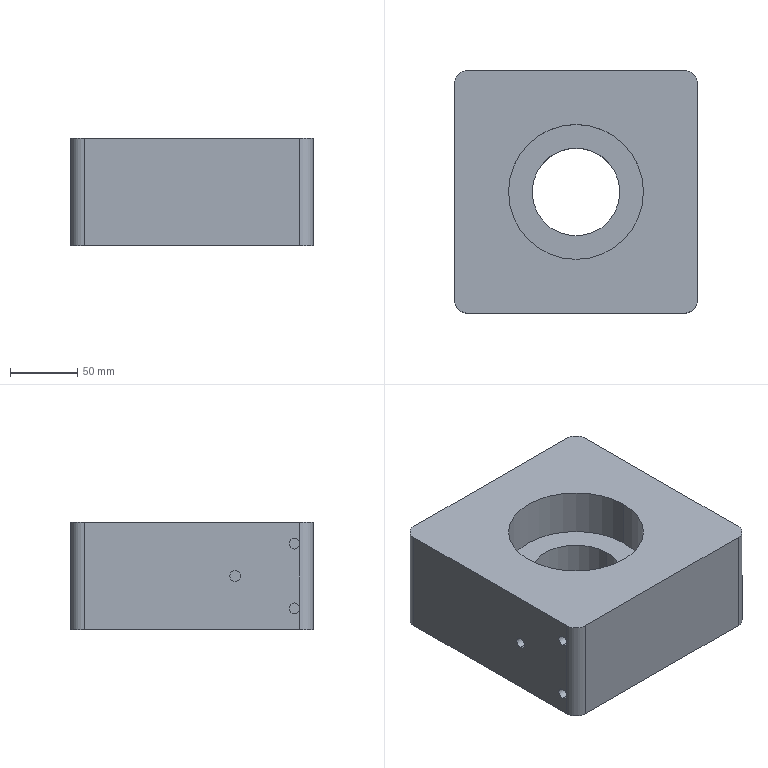Component | SolidWorks | CleaningRobotAssembly-1_FixingBlock-1 | 1 solid | 33 faces | box 180 x 180 x 80 mm | volume 2157904 mm3 | cylinder 20 | plane 13 | commonest cylinder face diameters 8 x12 20 x4 100 x2 65 x2
build123d program:
from build123d import *

# Parameters (mm, degrees)
SKETCH1_W           = 180
SKETCH1_H           = 180
BOSS_EXTRUDE1_DEPTH = 80
SKETCH2_R           = 32.5
CUT_EXTRUDE1_DEPTH  = 100
FILLET1_R           = 10
SKETCH3_R           = 4
CUT_EXTRUDE2_DEPTH  = 10
SKETCH4_R           = 50
CUT_EXTRUDE3_DEPTH  = 35


with BuildPart() as part:
    # Sketch1 → Boss-Extrude1 (new body)
    with BuildSketch(Plane.XY):
        Rectangle(SKETCH1_W, SKETCH1_H)
    extrude(amount=BOSS_EXTRUDE1_DEPTH)

    # Sketch2 → Cut-Extrude1 (cut)
    with BuildSketch(Plane(origin=(0, 0, 0), x_dir=(-1, 0, 0), z_dir=(0, 0, -1))):
        Circle(SKETCH2_R)
    extrude(amount=-CUT_EXTRUDE1_DEPTH, mode=Mode.SUBTRACT)

    # Fillet1
    fillet1_edges = [part.edges().sort_by_distance(p)[0] for p in [
        (-90, 90, 40),
        (90, 90, 40),
        (90, -90, 40),
        (-90, -90, 40),
    ]]
    fillet(fillet1_edges, radius=FILLET1_R)

    # Sketch3 → Cut-Extrude2 (cut)
    with BuildSketch(Plane(origin=(90, 0, 0), x_dir=(0, 0, -1), z_dir=(1, 0, 0))):
        with Locations((-16, 76)):
            Circle(SKETCH3_R)
        with Locations((-40, 32)):
            Circle(SKETCH3_R)
        with Locations((-64, 76)):
            Circle(SKETCH3_R)
    cut_extrude2 = extrude(amount=-CUT_EXTRUDE2_DEPTH, mode=Mode.SUBTRACT)

    # Mirror1: Cut-Extrude2 across plane
    add(cut_extrude2.mirror(Plane(origin=(0, 0, 0), x_dir=(0, 0, 1), z_dir=(1, 0, 0))), mode=Mode.SUBTRACT)

    # Sketch4 → Cut-Extrude3 (cut)
    with BuildSketch(Plane(origin=(0, 0, 0), x_dir=(-1, 0, 0), z_dir=(0, 0, -1))):
        Circle(SKETCH4_R)
    extrude(amount=-CUT_EXTRUDE3_DEPTH, mode=Mode.SUBTRACT)


solid = part.part

# Placed as in the assembly
solid = solid.moved(Location((310.629, 34.1, 268), (180, 0, 0)))
STEP:
#1=COLOUR_RGB('',0.7922,0.8196,0.9333);
#2=FILL_AREA_STYLE_COLOUR('',#1);
#3=FILL_AREA_STYLE('',(#2));
#4=SURFACE_STYLE_FILL_AREA(#3);
#5=SURFACE_SIDE_STYLE('',(#4));
#6=SURFACE_STYLE_USAGE(.BOTH.,#5);
#7=PRESENTATION_STYLE_ASSIGNMENT((#6));
#8=CARTESIAN_POINT('',(14.198,1.343,9.173));
#9=VERTEX_POINT('',#8);
#10=CARTESIAN_POINT('',(10.261,1.343,9.173));
#11=VERTEX_POINT('',#10);
#12=CARTESIAN_POINT('',(12.23,1.343,9.173));
#13=DIRECTION('',(0.,0.,1.));
#14=DIRECTION('',(-1.,-0.,0.));
#15=AXIS2_PLACEMENT_3D('',#12,#13,#14);
#16=CIRCLE('',#15,1.969);
#17=EDGE_CURVE('',#9,#11,#16,.T.);
#18=ORIENTED_EDGE('',*,*,#17,.F.);
#19=CARTESIAN_POINT('',(14.198,1.343,10.551));
#20=VERTEX_POINT('',#19);
#21=CARTESIAN_POINT('',(14.198,1.343,9.173));
#22=DIRECTION('',(0.,0.,1.));
#23=VECTOR('',#22,39.37);
#24=LINE('',#21,#23);
#25=EDGE_CURVE('',#9,#20,#24,.T.);
#26=ORIENTED_EDGE('',*,*,#25,.T.);
#27=CARTESIAN_POINT('',(10.261,1.343,10.551));
#28=VERTEX_POINT('',#27);
#29=CARTESIAN_POINT('',(12.23,1.343,10.551));
#30=DIRECTION('',(0.,0.,1.));
#31=DIRECTION('',(-1.,-0.,0.));
#32=AXIS2_PLACEMENT_3D('',#29,#30,#31);
#33=CIRCLE('',#32,1.969);
#34=EDGE_CURVE('',#20,#28,#33,.T.);
#35=ORIENTED_EDGE('',*,*,#34,.T.);
#36=CARTESIAN_POINT('',(10.261,1.343,9.173));
#37=DIRECTION('',(0.,0.,1.));
#38=VECTOR('',#37,39.37);
#39=LINE('',#36,#38);
#40=EDGE_CURVE('',#11,#28,#39,.T.);
#41=ORIENTED_EDGE('',*,*,#40,.F.);
#42=EDGE_LOOP('',(#18,#26,#35,#41));
#43=FACE_OUTER_BOUND('',#42,.T.);
#44=CARTESIAN_POINT('',(12.23,1.343,9.173));
#45=DIRECTION('',(0.,0.,1.));
#46=DIRECTION('',(-1.,-0.,0.));
#47=AXIS2_PLACEMENT_3D('',#44,#45,#46);
#48=CYLINDRICAL_SURFACE('',#47,1.969);
#49=ADVANCED_FACE('',(#43),#48,.F.);
#50=CARTESIAN_POINT('',(9.08,-1.65,9.764));
#51=VERTEX_POINT('',#50);
#52=CARTESIAN_POINT('',(9.08,-1.65,10.079));
#53=VERTEX_POINT('',#52);
#54=CARTESIAN_POINT('',(9.08,-1.65,9.921));
#55=DIRECTION('',(1.,0.,-0.));
#56=DIRECTION('',(0.,0.,1.));
#57=AXIS2_PLACEMENT_3D('',#54,#55,#56);
#58=CIRCLE('',#57,0.1575);
#59=EDGE_CURVE('',#51,#53,#58,.T.);
#60=ORIENTED_EDGE('',*,*,#59,.T.);
#61=CARTESIAN_POINT('',(8.686,-1.65,10.079));
#62=VERTEX_POINT('',#61);
#63=CARTESIAN_POINT('',(9.08,-1.65,10.079));
#64=DIRECTION('',(-1.,-0.,0.));
#65=VECTOR('',#64,39.37);
#66=LINE('',#63,#65);
#67=EDGE_CURVE('',#53,#62,#66,.T.);
#68=ORIENTED_EDGE('',*,*,#67,.T.);
#69=CARTESIAN_POINT('',(8.686,-1.65,9.764));
#70=VERTEX_POINT('',#69);
#71=CARTESIAN_POINT('',(8.686,-1.65,9.921));
#72=DIRECTION('',(1.,0.,-0.));
#73=DIRECTION('',(0.,0.,1.));
#74=AXIS2_PLACEMENT_3D('',#71,#72,#73);
#75=CIRCLE('',#74,0.1575);
#76=EDGE_CURVE('',#70,#62,#75,.T.);
#77=ORIENTED_EDGE('',*,*,#76,.F.);
#78=CARTESIAN_POINT('',(9.08,-1.65,9.764));
#79=DIRECTION('',(-1.,-0.,0.));
#80=VECTOR('',#79,39.37);
#81=LINE('',#78,#80);
#82=EDGE_CURVE('',#51,#70,#81,.T.);
#83=ORIENTED_EDGE('',*,*,#82,.F.);
#84=EDGE_LOOP('',(#60,#68,#77,#83));
#85=FACE_OUTER_BOUND('',#84,.T.);
#86=CARTESIAN_POINT('',(9.08,-1.65,9.921));
#87=DIRECTION('',(-1.,-0.,0.));
#88=DIRECTION('',(0.,0.,-1.));
#89=AXIS2_PLACEMENT_3D('',#86,#87,#88);
#90=CYLINDRICAL_SURFACE('',#89,0.1575);
#91=ADVANCED_FACE('',(#85),#90,.F.);
#92=CARTESIAN_POINT('',(9.08,0.08267,8.819));
#93=VERTEX_POINT('',#92);
#94=CARTESIAN_POINT('',(9.08,0.08267,9.134));
#95=VERTEX_POINT('',#94);
#96=CARTESIAN_POINT('',(9.08,0.08267,8.976));
#97=DIRECTION('',(1.,0.,-0.));
#98=DIRECTION('',(0.,0.,1.));
#99=AXIS2_PLACEMENT_3D('',#96,#97,#98);
#100=CIRCLE('',#99,0.1575);
#101=EDGE_CURVE('',#93,#95,#100,.T.);
#102=ORIENTED_EDGE('',*,*,#101,.T.);
#103=CARTESIAN_POINT('',(8.686,0.08267,9.134));
#104=VERTEX_POINT('',#103);
#105=CARTESIAN_POINT('',(9.08,0.08267,9.134));
#106=DIRECTION('',(-1.,-0.,0.));
#107=VECTOR('',#106,39.37);
#108=LINE('',#105,#107);
#109=EDGE_CURVE('',#95,#104,#108,.T.);
#110=ORIENTED_EDGE('',*,*,#109,.T.);
#111=CARTESIAN_POINT('',(8.686,0.08267,8.819));
#112=VERTEX_POINT('',#111);
#113=CARTESIAN_POINT('',(8.686,0.08267,8.976));
#114=DIRECTION('',(1.,0.,-0.));
#115=DIRECTION('',(0.,0.,1.));
#116=AXIS2_PLACEMENT_3D('',#113,#114,#115);
#117=CIRCLE('',#116,0.1575);
#118=EDGE_CURVE('',#112,#104,#117,.T.);
#119=ORIENTED_EDGE('',*,*,#118,.F.);
#120=CARTESIAN_POINT('',(9.08,0.08267,8.819));
#121=DIRECTION('',(-1.,-0.,0.));
#122=VECTOR('',#121,39.37);
#123=LINE('',#120,#122);
#124=EDGE_CURVE('',#93,#112,#123,.T.);
#125=ORIENTED_EDGE('',*,*,#124,.F.);
#126=EDGE_LOOP('',(#102,#110,#119,#125));
#127=FACE_OUTER_BOUND('',#126,.T.);
#128=CARTESIAN_POINT('',(9.08,0.08267,8.976));
#129=DIRECTION('',(-1.,-0.,0.));
#130=DIRECTION('',(0.,0.,-1.));
#131=AXIS2_PLACEMENT_3D('',#128,#129,#130);
#132=CYLINDRICAL_SURFACE('',#131,0.1575);
#133=ADVANCED_FACE('',(#127),#132,.F.);
#134=CARTESIAN_POINT('',(9.08,-1.65,7.874));
#135=VERTEX_POINT('',#134);
#136=CARTESIAN_POINT('',(9.08,-1.65,8.189));
#137=VERTEX_POINT('',#136);
#138=CARTESIAN_POINT('',(9.08,-1.65,8.031));
#139=DIRECTION('',(1.,0.,-0.));
#140=DIRECTION('',(0.,0.,1.));
#141=AXIS2_PLACEMENT_3D('',#138,#139,#140);
#142=CIRCLE('',#141,0.1575);
#143=EDGE_CURVE('',#135,#137,#142,.T.);
#144=ORIENTED_EDGE('',*,*,#143,.T.);
#145=CARTESIAN_POINT('',(8.686,-1.65,8.189));
#146=VERTEX_POINT('',#145);
#147=CARTESIAN_POINT('',(9.08,-1.65,8.189));
#148=DIRECTION('',(-1.,-0.,0.));
#149=VECTOR('',#148,39.37);
#150=LINE('',#147,#149);
#151=EDGE_CURVE('',#137,#146,#150,.T.);
#152=ORIENTED_EDGE('',*,*,#151,.T.);
#153=CARTESIAN_POINT('',(8.686,-1.65,7.874));
#154=VERTEX_POINT('',#153);
#155=CARTESIAN_POINT('',(8.686,-1.65,8.031));
#156=DIRECTION('',(1.,0.,-0.));
#157=DIRECTION('',(0.,0.,1.));
#158=AXIS2_PLACEMENT_3D('',#155,#156,#157);
#159=CIRCLE('',#158,0.1575);
#160=EDGE_CURVE('',#154,#146,#159,.T.);
#161=ORIENTED_EDGE('',*,*,#160,.F.);
#162=CARTESIAN_POINT('',(9.08,-1.65,7.874));
#163=DIRECTION('',(-1.,-0.,0.));
#164=VECTOR('',#163,39.37);
#165=LINE('',#162,#164);
#166=EDGE_CURVE('',#135,#154,#165,.T.);
#167=ORIENTED_EDGE('',*,*,#166,.F.);
#168=EDGE_LOOP('',(#144,#152,#161,#167));
#169=FACE_OUTER_BOUND('',#168,.T.);
#170=CARTESIAN_POINT('',(9.08,-1.65,8.031));
#171=DIRECTION('',(-1.,-0.,0.));
#172=DIRECTION('',(0.,0.,-1.));
#173=AXIS2_PLACEMENT_3D('',#170,#171,#172);
#174=CYLINDRICAL_SURFACE('',#173,0.1575);
#175=ADVANCED_FACE('',(#169),#174,.F.);
#176=CARTESIAN_POINT('',(15.379,-1.65,9.764));
#177=VERTEX_POINT('',#176);
#178=CARTESIAN_POINT('',(15.379,-1.65,10.079));
#179=VERTEX_POINT('',#178);
#180=CARTESIAN_POINT('',(15.379,-1.65,9.921));
#181=DIRECTION('',(1.,0.,-0.));
#182=DIRECTION('',(0.,0.,1.));
#183=AXIS2_PLACEMENT_3D('',#180,#181,#182);
#184=CIRCLE('',#183,0.1575);
#185=EDGE_CURVE('',#177,#179,#184,.T.);
#186=ORIENTED_EDGE('',*,*,#185,.F.);
#187=CARTESIAN_POINT('',(15.773,-1.65,9.764));
#188=VERTEX_POINT('',#187);
#189=CARTESIAN_POINT('',(15.379,-1.65,9.764));
#190=DIRECTION('',(1.,0.,-0.));
#191=VECTOR('',#190,39.37);
#192=LINE('',#189,#191);
#193=EDGE_CURVE('',#177,#188,#192,.T.);
#194=ORIENTED_EDGE('',*,*,#193,.T.);
#195=CARTESIAN_POINT('',(15.773,-1.65,10.079));
#196=VERTEX_POINT('',#195);
#197=CARTESIAN_POINT('',(15.773,-1.65,9.921));
#198=DIRECTION('',(1.,0.,-0.));
#199=DIRECTION('',(0.,0.,1.));
#200=AXIS2_PLACEMENT_3D('',#197,#198,#199);
#201=CIRCLE('',#200,0.1575);
#202=EDGE_CURVE('',#188,#196,#201,.T.);
#203=ORIENTED_EDGE('',*,*,#202,.T.);
#204=CARTESIAN_POINT('',(15.379,-1.65,10.079));
#205=DIRECTION('',(1.,0.,-0.));
#206=VECTOR('',#205,39.37);
#207=LINE('',#204,#206);
#208=EDGE_CURVE('',#179,#196,#207,.T.);
#209=ORIENTED_EDGE('',*,*,#208,.F.);
#210=EDGE_LOOP('',(#186,#194,#203,#209));
#211=FACE_OUTER_BOUND('',#210,.T.);
#212=CARTESIAN_POINT('',(15.379,-1.65,9.921));
#213=DIRECTION('',(1.,0.,-0.));
#214=DIRECTION('',(0.,0.,1.));
#215=AXIS2_PLACEMENT_3D('',#212,#213,#214);
#216=CYLINDRICAL_SURFACE('',#215,0.1575);
#217=ADVANCED_FACE('',(#211),#216,.F.);
#218=CARTESIAN_POINT('',(15.379,0.08267,8.819));
#219=VERTEX_POINT('',#218);
#220=CARTESIAN_POINT('',(15.379,0.08267,9.134));
#221=VERTEX_POINT('',#220);
#222=CARTESIAN_POINT('',(15.379,0.08267,8.976));
#223=DIRECTION('',(1.,0.,-0.));
#224=DIRECTION('',(0.,0.,1.));
#225=AXIS2_PLACEMENT_3D('',#222,#223,#224);
#226=CIRCLE('',#225,0.1575);
#227=EDGE_CURVE('',#219,#221,#226,.T.);
#228=ORIENTED_EDGE('',*,*,#227,.F.);
#229=CARTESIAN_POINT('',(15.773,0.08267,8.819));
#230=VERTEX_POINT('',#229);
#231=CARTESIAN_POINT('',(15.379,0.08267,8.819));
#232=DIRECTION('',(1.,0.,-0.));
#233=VECTOR('',#232,39.37);
#234=LINE('',#231,#233);
#235=EDGE_CURVE('',#219,#230,#234,.T.);
#236=ORIENTED_EDGE('',*,*,#235,.T.);
#237=CARTESIAN_POINT('',(15.773,0.08267,9.134));
#238=VERTEX_POINT('',#237);
#239=CARTESIAN_POINT('',(15.773,0.08267,8.976));
#240=DIRECTION('',(1.,0.,-0.));
#241=DIRECTION('',(0.,0.,1.));
#242=AXIS2_PLACEMENT_3D('',#239,#240,#241);
#243=CIRCLE('',#242,0.1575);
#244=EDGE_CURVE('',#230,#238,#243,.T.);
#245=ORIENTED_EDGE('',*,*,#244,.T.);
#246=CARTESIAN_POINT('',(15.379,0.08267,9.134));
#247=DIRECTION('',(1.,0.,-0.));
#248=VECTOR('',#247,39.37);
#249=LINE('',#246,#248);
#250=EDGE_CURVE('',#221,#238,#249,.T.);
#251=ORIENTED_EDGE('',*,*,#250,.F.);
#252=EDGE_LOOP('',(#228,#236,#245,#251));
#253=FACE_OUTER_BOUND('',#252,.T.);
#254=CARTESIAN_POINT('',(15.379,0.08267,8.976));
#255=DIRECTION('',(1.,0.,-0.));
#256=DIRECTION('',(0.,0.,1.));
#257=AXIS2_PLACEMENT_3D('',#254,#255,#256);
#258=CYLINDRICAL_SURFACE('',#257,0.1575);
#259=ADVANCED_FACE('',(#253),#258,.F.);
#260=CARTESIAN_POINT('',(15.379,-1.65,7.874));
#261=VERTEX_POINT('',#260);
#262=CARTESIAN_POINT('',(15.379,-1.65,8.189));
#263=VERTEX_POINT('',#262);
#264=CARTESIAN_POINT('',(15.379,-1.65,8.031));
#265=DIRECTION('',(1.,0.,-0.));
#266=DIRECTION('',(0.,0.,1.));
#267=AXIS2_PLACEMENT_3D('',#264,#265,#266);
#268=CIRCLE('',#267,0.1575);
#269=EDGE_CURVE('',#261,#263,#268,.T.);
#270=ORIENTED_EDGE('',*,*,#269,.F.);
#271=CARTESIAN_POINT('',(15.773,-1.65,7.874));
#272=VERTEX_POINT('',#271);
#273=CARTESIAN_POINT('',(15.379,-1.65,7.874));
#274=DIRECTION('',(1.,0.,-0.));
#275=VECTOR('',#274,39.37);
#276=LINE('',#273,#275);
#277=EDGE_CURVE('',#261,#272,#276,.T.);
#278=ORIENTED_EDGE('',*,*,#277,.T.);
#279=CARTESIAN_POINT('',(15.773,-1.65,8.189));
#280=VERTEX_POINT('',#279);
#281=CARTESIAN_POINT('',(15.773,-1.65,8.031));
#282=DIRECTION('',(1.,0.,-0.));
#283=DIRECTION('',(0.,0.,1.));
#284=AXIS2_PLACEMENT_3D('',#281,#282,#283);
#285=CIRCLE('',#284,0.1575);
#286=EDGE_CURVE('',#272,#280,#285,.T.);
#287=ORIENTED_EDGE('',*,*,#286,.T.);
#288=CARTESIAN_POINT('',(15.379,-1.65,8.189));
#289=DIRECTION('',(1.,0.,-0.));
#290=VECTOR('',#289,39.37);
#291=LINE('',#288,#290);
#292=EDGE_CURVE('',#263,#280,#291,.T.);
#293=ORIENTED_EDGE('',*,*,#292,.F.);
#294=EDGE_LOOP('',(#270,#278,#287,#293));
#295=FACE_OUTER_BOUND('',#294,.T.);
#296=CARTESIAN_POINT('',(15.379,-1.65,8.031));
#297=DIRECTION('',(1.,0.,-0.));
#298=DIRECTION('',(0.,0.,1.));
#299=AXIS2_PLACEMENT_3D('',#296,#297,#298);
#300=CYLINDRICAL_SURFACE('',#299,0.1575);
#301=ADVANCED_FACE('',(#295),#300,.F.);
#302=CARTESIAN_POINT('',(10.95,1.343,7.402));
#303=VERTEX_POINT('',#302);
#304=CARTESIAN_POINT('',(13.509,1.343,7.402));
#305=VERTEX_POINT('',#304);
#306=CARTESIAN_POINT('',(12.23,1.343,7.402));
#307=DIRECTION('',(-0.,-0.,-1.));
#308=DIRECTION('',(1.,0.,0.));
#309=AXIS2_PLACEMENT_3D('',#306,#307,#308);
#310=CIRCLE('',#309,1.28);
#311=EDGE_CURVE('',#303,#305,#310,.T.);
#312=ORIENTED_EDGE('',*,*,#311,.T.);
#313=CARTESIAN_POINT('',(13.509,1.343,9.173));
#314=VERTEX_POINT('',#313);
#315=CARTESIAN_POINT('',(13.509,1.343,6.614));
#316=DIRECTION('',(0.,0.,1.));
#317=VECTOR('',#316,39.37);
#318=LINE('',#315,#317);
#319=EDGE_CURVE('',#305,#314,#318,.T.);
#320=ORIENTED_EDGE('',*,*,#319,.T.);
#321=CARTESIAN_POINT('',(10.95,1.343,9.173));
#322=VERTEX_POINT('',#321);
#323=CARTESIAN_POINT('',(12.23,1.343,9.173));
#324=DIRECTION('',(-0.,-0.,-1.));
#325=DIRECTION('',(-1.,-0.,0.));
#326=AXIS2_PLACEMENT_3D('',#323,#324,#325);
#327=CIRCLE('',#326,1.28);
#328=EDGE_CURVE('',#322,#314,#327,.T.);
#329=ORIENTED_EDGE('',*,*,#328,.F.);
#330=CARTESIAN_POINT('',(10.95,1.343,6.614));
#331=DIRECTION('',(0.,0.,1.));
#332=VECTOR('',#331,39.37);
#333=LINE('',#330,#332);
#334=EDGE_CURVE('',#303,#322,#333,.T.);
#335=ORIENTED_EDGE('',*,*,#334,.F.);
#336=EDGE_LOOP('',(#312,#320,#329,#335));
#337=FACE_OUTER_BOUND('',#336,.T.);
#338=CARTESIAN_POINT('',(12.23,1.343,6.614));
#339=DIRECTION('',(0.,0.,1.));
#340=DIRECTION('',(-1.,-0.,0.));
#341=AXIS2_PLACEMENT_3D('',#338,#339,#340);
#342=CYLINDRICAL_SURFACE('',#341,1.28);
#343=ADVANCED_FACE('',(#337),#342,.F.);
#344=ORIENTED_EDGE('',*,*,#319,.F.);
#345=CARTESIAN_POINT('',(12.23,1.343,7.402));
#346=DIRECTION('',(-0.,-0.,-1.));
#347=DIRECTION('',(1.,0.,0.));
#348=AXIS2_PLACEMENT_3D('',#345,#346,#347);
#349=CIRCLE('',#348,1.28);
#350=EDGE_CURVE('',#305,#303,#349,.T.);
#351=ORIENTED_EDGE('',*,*,#350,.T.);
#352=ORIENTED_EDGE('',*,*,#334,.T.);
#353=CARTESIAN_POINT('',(12.23,1.343,9.173));
#354=DIRECTION('',(-0.,-0.,-1.));
#355=DIRECTION('',(-1.,-0.,0.));
#356=AXIS2_PLACEMENT_3D('',#353,#354,#355);
#357=CIRCLE('',#356,1.28);
#358=EDGE_CURVE('',#314,#322,#357,.T.);
#359=ORIENTED_EDGE('',*,*,#358,.F.);
#360=EDGE_LOOP('',(#344,#351,#352,#359));
#361=FACE_OUTER_BOUND('',#360,.T.);
#362=CARTESIAN_POINT('',(12.23,1.343,6.614));
#363=DIRECTION('',(0.,0.,1.));
#364=DIRECTION('',(-1.,-0.,0.));
#365=AXIS2_PLACEMENT_3D('',#362,#363,#364);
#366=CYLINDRICAL_SURFACE('',#365,1.28);
#367=ADVANCED_FACE('',(#361),#366,.F.);
#368=ORIENTED_EDGE('',*,*,#118,.T.);
#369=CARTESIAN_POINT('',(8.686,0.08267,8.976));
#370=DIRECTION('',(1.,0.,-0.));
#371=DIRECTION('',(0.,0.,1.));
#372=AXIS2_PLACEMENT_3D('',#369,#370,#371);
#373=CIRCLE('',#372,0.1575);
#374=EDGE_CURVE('',#104,#112,#373,.T.);
#375=ORIENTED_EDGE('',*,*,#374,.T.);
#376=EDGE_LOOP('',(#368,#375));
#377=FACE_BOUND('',#376,.T.);
#378=CARTESIAN_POINT('',(8.686,-1.807,8.031));
#379=VERTEX_POINT('',#378);
#380=CARTESIAN_POINT('',(8.686,-1.807,9.921));
#381=VERTEX_POINT('',#380);
#382=CARTESIAN_POINT('',(8.686,-1.807,7.402));
#383=DIRECTION('',(0.,0.,1.));
#384=VECTOR('',#383,39.37);
#385=LINE('',#382,#384);
#386=EDGE_CURVE('',#379,#381,#385,.T.);
#387=ORIENTED_EDGE('',*,*,#386,.T.);
#388=CARTESIAN_POINT('',(8.686,-1.65,9.921));
#389=DIRECTION('',(1.,0.,-0.));
#390=DIRECTION('',(0.,0.,1.));
#391=AXIS2_PLACEMENT_3D('',#388,#389,#390);
#392=CIRCLE('',#391,0.1575);
#393=EDGE_CURVE('',#381,#70,#392,.T.);
#394=ORIENTED_EDGE('',*,*,#393,.T.);
#395=ORIENTED_EDGE('',*,*,#76,.T.);
#396=CARTESIAN_POINT('',(8.686,-1.65,9.921));
#397=DIRECTION('',(1.,0.,-0.));
#398=DIRECTION('',(0.,0.,1.));
#399=AXIS2_PLACEMENT_3D('',#396,#397,#398);
#400=CIRCLE('',#399,0.1575);
#401=EDGE_CURVE('',#62,#381,#400,.T.);
#402=ORIENTED_EDGE('',*,*,#401,.T.);
#403=CARTESIAN_POINT('',(8.686,-1.807,10.551));
#404=VERTEX_POINT('',#403);
#405=CARTESIAN_POINT('',(8.686,-1.807,7.402));
#406=DIRECTION('',(0.,0.,1.));
#407=VECTOR('',#406,39.37);
#408=LINE('',#405,#407);
#409=EDGE_CURVE('',#381,#404,#408,.T.);
#410=ORIENTED_EDGE('',*,*,#409,.T.);
#411=CARTESIAN_POINT('',(8.686,4.492,10.551));
#412=VERTEX_POINT('',#411);
#413=CARTESIAN_POINT('',(8.686,4.886,10.551));
#414=DIRECTION('',(-0.,1.,-0.));
#415=VECTOR('',#414,39.37);
#416=LINE('',#413,#415);
#417=EDGE_CURVE('',#404,#412,#416,.T.);
#418=ORIENTED_EDGE('',*,*,#417,.T.);
#419=CARTESIAN_POINT('',(8.686,4.492,7.402));
#420=VERTEX_POINT('',#419);
#421=CARTESIAN_POINT('',(8.686,4.492,7.402));
#422=DIRECTION('',(-0.,-0.,-1.));
#423=VECTOR('',#422,39.37);
#424=LINE('',#421,#423);
#425=EDGE_CURVE('',#412,#420,#424,.T.);
#426=ORIENTED_EDGE('',*,*,#425,.T.);
#427=CARTESIAN_POINT('',(8.686,-1.807,7.402));
#428=VERTEX_POINT('',#427);
#429=CARTESIAN_POINT('',(8.686,4.886,7.402));
#430=DIRECTION('',(-0.,1.,-0.));
#431=VECTOR('',#430,39.37);
#432=LINE('',#429,#431);
#433=EDGE_CURVE('',#428,#420,#432,.T.);
#434=ORIENTED_EDGE('',*,*,#433,.F.);
#435=CARTESIAN_POINT('',(8.686,-1.807,7.402));
#436=DIRECTION('',(0.,0.,1.));
#437=VECTOR('',#436,39.37);
#438=LINE('',#435,#437);
#439=EDGE_CURVE('',#428,#379,#438,.T.);
#440=ORIENTED_EDGE('',*,*,#439,.T.);
#441=CARTESIAN_POINT('',(8.686,-1.65,8.031));
#442=DIRECTION('',(1.,0.,-0.));
#443=DIRECTION('',(0.,0.,1.));
#444=AXIS2_PLACEMENT_3D('',#441,#442,#443);
#445=CIRCLE('',#444,0.1575);
#446=EDGE_CURVE('',#379,#154,#445,.T.);
#447=ORIENTED_EDGE('',*,*,#446,.T.);
#448=ORIENTED_EDGE('',*,*,#160,.T.);
#449=CARTESIAN_POINT('',(8.686,-1.65,8.031));
#450=DIRECTION('',(1.,0.,-0.));
#451=DIRECTION('',(0.,0.,1.));
#452=AXIS2_PLACEMENT_3D('',#449,#450,#451);
#453=CIRCLE('',#452,0.1575);
#454=EDGE_CURVE('',#146,#379,#453,.T.);
#455=ORIENTED_EDGE('',*,*,#454,.T.);
#456=EDGE_LOOP('',(#387,#394,#395,#402,#410,#418,#426,#434,#440,#447,#448,#455));
#457=FACE_OUTER_BOUND('',#456,.T.);
#458=CARTESIAN_POINT('',(8.686,4.886,7.402));
#459=DIRECTION('',(1.,0.,-0.));
#460=DIRECTION('',(0.,0.,1.));
#461=AXIS2_PLACEMENT_3D('',#458,#459,#460);
#462=PLANE('',#461);
#463=ADVANCED_FACE('',(#377,#457),#462,.F.);
#464=CARTESIAN_POINT('',(9.08,4.886,7.402));
#465=VERTEX_POINT('',#464);
#466=CARTESIAN_POINT('',(15.379,4.886,7.402));
#467=VERTEX_POINT('',#466);
#468=CARTESIAN_POINT('',(15.773,4.886,7.402));
#469=DIRECTION('',(1.,0.,-0.));
#470=VECTOR('',#469,39.37);
#471=LINE('',#468,#470);
#472=EDGE_CURVE('',#465,#467,#471,.T.);
#473=ORIENTED_EDGE('',*,*,#472,.F.);
#474=CARTESIAN_POINT('',(9.08,4.886,10.551));
#475=VERTEX_POINT('',#474);
#476=CARTESIAN_POINT('',(9.08,4.886,7.402));
#477=DIRECTION('',(0.,0.,1.));
#478=VECTOR('',#477,39.37);
#479=LINE('',#476,#478);
#480=EDGE_CURVE('',#465,#475,#479,.T.);
#481=ORIENTED_EDGE('',*,*,#480,.T.);
#482=CARTESIAN_POINT('',(15.379,4.886,10.551));
#483=VERTEX_POINT('',#482);
#484=CARTESIAN_POINT('',(15.773,4.886,10.551));
#485=DIRECTION('',(1.,0.,-0.));
#486=VECTOR('',#485,39.37);
#487=LINE('',#484,#486);
#488=EDGE_CURVE('',#475,#483,#487,.T.);
#489=ORIENTED_EDGE('',*,*,#488,.T.);
#490=CARTESIAN_POINT('',(15.379,4.886,7.402));
#491=DIRECTION('',(-0.,-0.,-1.));
#492=VECTOR('',#491,39.37);
#493=LINE('',#490,#492);
#494=EDGE_CURVE('',#483,#467,#493,.T.);
#495=ORIENTED_EDGE('',*,*,#494,.T.);
#496=EDGE_LOOP('',(#473,#481,#489,#495));
#497=FACE_OUTER_BOUND('',#496,.T.);
#498=CARTESIAN_POINT('',(15.773,4.886,7.402));
#499=DIRECTION('',(0.,-1.,0.));
#500=DIRECTION('',(-1.,-0.,0.));
#501=AXIS2_PLACEMENT_3D('',#498,#499,#500);
#502=PLANE('',#501);
#503=ADVANCED_FACE('',(#497),#502,.F.);
#504=CARTESIAN_POINT('',(15.773,0.08267,8.976));
#505=DIRECTION('',(1.,0.,-0.));
#506=DIRECTION('',(0.,0.,1.));
#507=AXIS2_PLACEMENT_3D('',#504,#505,#506);
#508=CIRCLE('',#507,0.1575);
#509=EDGE_CURVE('',#238,#230,#508,.T.);
#510=ORIENTED_EDGE('',*,*,#509,.F.);
#511=ORIENTED_EDGE('',*,*,#244,.F.);
#512=EDGE_LOOP('',(#510,#511));
#513=FACE_BOUND('',#512,.T.);
#514=CARTESIAN_POINT('',(15.773,-1.807,10.551));
#515=VERTEX_POINT('',#514);
#516=CARTESIAN_POINT('',(15.773,-1.807,9.921));
#517=VERTEX_POINT('',#516);
#518=CARTESIAN_POINT('',(15.773,-1.807,7.402));
#519=DIRECTION('',(-0.,-0.,-1.));
#520=VECTOR('',#519,39.37);
#521=LINE('',#518,#520);
#522=EDGE_CURVE('',#515,#517,#521,.T.);
#523=ORIENTED_EDGE('',*,*,#522,.T.);
#524=CARTESIAN_POINT('',(15.773,-1.65,9.921));
#525=DIRECTION('',(1.,0.,-0.));
#526=DIRECTION('',(0.,0.,1.));
#527=AXIS2_PLACEMENT_3D('',#524,#525,#526);
#528=CIRCLE('',#527,0.1575);
#529=EDGE_CURVE('',#196,#517,#528,.T.);
#530=ORIENTED_EDGE('',*,*,#529,.F.);
#531=ORIENTED_EDGE('',*,*,#202,.F.);
#532=CARTESIAN_POINT('',(15.773,-1.65,9.921));
#533=DIRECTION('',(1.,0.,-0.));
#534=DIRECTION('',(0.,0.,1.));
#535=AXIS2_PLACEMENT_3D('',#532,#533,#534);
#536=CIRCLE('',#535,0.1575);
#537=EDGE_CURVE('',#517,#188,#536,.T.);
#538=ORIENTED_EDGE('',*,*,#537,.F.);
#539=CARTESIAN_POINT('',(15.773,-1.807,8.031));
#540=VERTEX_POINT('',#539);
#541=CARTESIAN_POINT('',(15.773,-1.807,7.402));
#542=DIRECTION('',(-0.,-0.,-1.));
#543=VECTOR('',#542,39.37);
#544=LINE('',#541,#543);
#545=EDGE_CURVE('',#517,#540,#544,.T.);
#546=ORIENTED_EDGE('',*,*,#545,.T.);
#547=CARTESIAN_POINT('',(15.773,-1.65,8.031));
#548=DIRECTION('',(1.,0.,-0.));
#549=DIRECTION('',(0.,0.,1.));
#550=AXIS2_PLACEMENT_3D('',#547,#548,#549);
#551=CIRCLE('',#550,0.1575);
#552=EDGE_CURVE('',#280,#540,#551,.T.);
#553=ORIENTED_EDGE('',*,*,#552,.F.);
#554=ORIENTED_EDGE('',*,*,#286,.F.);
#555=CARTESIAN_POINT('',(15.773,-1.65,8.031));
#556=DIRECTION('',(1.,0.,-0.));
#557=DIRECTION('',(0.,0.,1.));
#558=AXIS2_PLACEMENT_3D('',#555,#556,#557);
#559=CIRCLE('',#558,0.1575);
#560=EDGE_CURVE('',#540,#272,#559,.T.);
#561=ORIENTED_EDGE('',*,*,#560,.F.);
#562=CARTESIAN_POINT('',(15.773,-1.807,7.402));
#563=VERTEX_POINT('',#562);
#564=CARTESIAN_POINT('',(15.773,-1.807,7.402));
#565=DIRECTION('',(-0.,-0.,-1.));
#566=VECTOR('',#565,39.37);
#567=LINE('',#564,#566);
#568=EDGE_CURVE('',#540,#563,#567,.T.);
#569=ORIENTED_EDGE('',*,*,#568,.T.);
#570=CARTESIAN_POINT('',(15.773,4.492,7.402));
#571=VERTEX_POINT('',#570);
#572=CARTESIAN_POINT('',(15.773,4.886,7.402));
#573=DIRECTION('',(0.,-1.,0.));
#574=VECTOR('',#573,39.37);
#575=LINE('',#572,#574);
#576=EDGE_CURVE('',#571,#563,#575,.T.);
#577=ORIENTED_EDGE('',*,*,#576,.F.);
#578=CARTESIAN_POINT('',(15.773,4.492,10.551));
#579=VERTEX_POINT('',#578);
#580=CARTESIAN_POINT('',(15.773,4.492,7.402));
#581=DIRECTION('',(0.,0.,1.));
#582=VECTOR('',#581,39.37);
#583=LINE('',#580,#582);
#584=EDGE_CURVE('',#571,#579,#583,.T.);
#585=ORIENTED_EDGE('',*,*,#584,.T.);
#586=CARTESIAN_POINT('',(15.773,4.886,10.551));
#587=DIRECTION('',(0.,-1.,0.));
#588=VECTOR('',#587,39.37);
#589=LINE('',#586,#588);
#590=EDGE_CURVE('',#579,#515,#589,.T.);
#591=ORIENTED_EDGE('',*,*,#590,.T.);
#592=EDGE_LOOP('',(#523,#530,#531,#538,#546,#553,#554,#561,#569,#577,#585,#591));
#593=FACE_OUTER_BOUND('',#592,.T.);
#594=CARTESIAN_POINT('',(15.773,4.886,7.402));
#595=DIRECTION('',(-1.,-0.,0.));
#596=DIRECTION('',(-0.,-0.,-1.));
#597=AXIS2_PLACEMENT_3D('',#594,#595,#596);
#598=PLANE('',#597);
#599=ADVANCED_FACE('',(#513,#593),#598,.F.);
#600=CARTESIAN_POINT('',(15.379,-2.201,7.402));
#601=VERTEX_POINT('',#600);
#602=CARTESIAN_POINT('',(9.08,-2.201,7.402));
#603=VERTEX_POINT('',#602);
#604=CARTESIAN_POINT('',(15.773,-2.201,7.402));
#605=DIRECTION('',(-1.,-0.,0.));
#606=VECTOR('',#605,39.37);
#607=LINE('',#604,#606);
#608=EDGE_CURVE('',#601,#603,#607,.T.);
#609=ORIENTED_EDGE('',*,*,#608,.F.);
#610=CARTESIAN_POINT('',(15.379,-2.201,10.551));
#611=VERTEX_POINT('',#610);
#612=CARTESIAN_POINT('',(15.379,-2.201,7.402));
#613=DIRECTION('',(0.,0.,1.));
#614=VECTOR('',#613,39.37);
#615=LINE('',#612,#614);
#616=EDGE_CURVE('',#601,#611,#615,.T.);
#617=ORIENTED_EDGE('',*,*,#616,.T.);
#618=CARTESIAN_POINT('',(9.08,-2.201,10.551));
#619=VERTEX_POINT('',#618);
#620=CARTESIAN_POINT('',(15.773,-2.201,10.551));
#621=DIRECTION('',(-1.,-0.,0.));
#622=VECTOR('',#621,39.37);
#623=LINE('',#620,#622);
#624=EDGE_CURVE('',#611,#619,#623,.T.);
#625=ORIENTED_EDGE('',*,*,#624,.T.);
#626=CARTESIAN_POINT('',(9.08,-2.201,7.402));
#627=DIRECTION('',(-0.,-0.,-1.));
#628=VECTOR('',#627,39.37);
#629=LINE('',#626,#628);
#630=EDGE_CURVE('',#619,#603,#629,.T.);
#631=ORIENTED_EDGE('',*,*,#630,.T.);
#632=EDGE_LOOP('',(#609,#617,#625,#631));
#633=FACE_OUTER_BOUND('',#632,.T.);
#634=CARTESIAN_POINT('',(15.773,-2.201,7.402));
#635=DIRECTION('',(-0.,1.,-0.));
#636=DIRECTION('',(1.,0.,-0.));
#637=AXIS2_PLACEMENT_3D('',#634,#635,#636);
#638=PLANE('',#637);
#639=ADVANCED_FACE('',(#633),#638,.F.);
#640=ORIENTED_EDGE('',*,*,#311,.F.);
#641=ORIENTED_EDGE('',*,*,#350,.F.);
#642=EDGE_LOOP('',(#640,#641));
#643=FACE_BOUND('',#642,.T.);
#644=ORIENTED_EDGE('',*,*,#433,.T.);
#645=CARTESIAN_POINT('',(9.08,4.492,7.402));
#646=DIRECTION('',(-0.,-0.,-1.));
#647=DIRECTION('',(1.,0.,0.));
#648=AXIS2_PLACEMENT_3D('',#645,#646,#647);
#649=CIRCLE('',#648,0.3937);
#650=EDGE_CURVE('',#420,#465,#649,.T.);
#651=ORIENTED_EDGE('',*,*,#650,.T.);
#652=ORIENTED_EDGE('',*,*,#472,.T.);
#653=CARTESIAN_POINT('',(15.379,4.492,7.402));
#654=DIRECTION('',(-0.,-0.,-1.));
#655=DIRECTION('',(1.,0.,0.));
#656=AXIS2_PLACEMENT_3D('',#653,#654,#655);
#657=CIRCLE('',#656,0.3937);
#658=EDGE_CURVE('',#467,#571,#657,.T.);
#659=ORIENTED_EDGE('',*,*,#658,.T.);
#660=ORIENTED_EDGE('',*,*,#576,.T.);
#661=CARTESIAN_POINT('',(15.379,-1.807,7.402));
#662=DIRECTION('',(-0.,-0.,-1.));
#663=DIRECTION('',(1.,0.,0.));
#664=AXIS2_PLACEMENT_3D('',#661,#662,#663);
#665=CIRCLE('',#664,0.3937);
#666=EDGE_CURVE('',#563,#601,#665,.T.);
#667=ORIENTED_EDGE('',*,*,#666,.T.);
#668=ORIENTED_EDGE('',*,*,#608,.T.);
#669=CARTESIAN_POINT('',(9.08,-1.807,7.402));
#670=DIRECTION('',(-0.,-0.,-1.));
#671=DIRECTION('',(1.,0.,0.));
#672=AXIS2_PLACEMENT_3D('',#669,#670,#671);
#673=CIRCLE('',#672,0.3937);
#674=EDGE_CURVE('',#603,#428,#673,.T.);
#675=ORIENTED_EDGE('',*,*,#674,.T.);
#676=EDGE_LOOP('',(#644,#651,#652,#659,#660,#667,#668,#675));
#677=FACE_OUTER_BOUND('',#676,.T.);
#678=CARTESIAN_POINT('',(12.23,1.343,7.402));
#679=DIRECTION('',(-0.,-0.,-1.));
#680=DIRECTION('',(1.,0.,-0.));
#681=AXIS2_PLACEMENT_3D('',#678,#679,#680);
#682=PLANE('',#681);
#683=ADVANCED_FACE('',(#643,#677),#682,.T.);
#684=CARTESIAN_POINT('',(12.23,1.343,10.551));
#685=DIRECTION('',(0.,0.,1.));
#686=DIRECTION('',(-1.,-0.,0.));
#687=AXIS2_PLACEMENT_3D('',#684,#685,#686);
#688=CIRCLE('',#687,1.969);
#689=EDGE_CURVE('',#28,#20,#688,.T.);
#690=ORIENTED_EDGE('',*,*,#689,.F.);
#691=ORIENTED_EDGE('',*,*,#34,.F.);
#692=EDGE_LOOP('',(#690,#691));
#693=FACE_BOUND('',#692,.T.);
#694=ORIENTED_EDGE('',*,*,#488,.F.);
#695=CARTESIAN_POINT('',(9.08,4.492,10.551));
#696=DIRECTION('',(0.,0.,1.));
#697=DIRECTION('',(1.,0.,0.));
#698=AXIS2_PLACEMENT_3D('',#695,#696,#697);
#699=CIRCLE('',#698,0.3937);
#700=EDGE_CURVE('',#475,#412,#699,.T.);
#701=ORIENTED_EDGE('',*,*,#700,.T.);
#702=ORIENTED_EDGE('',*,*,#417,.F.);
#703=CARTESIAN_POINT('',(9.08,-1.807,10.551));
#704=DIRECTION('',(0.,0.,1.));
#705=DIRECTION('',(1.,0.,0.));
#706=AXIS2_PLACEMENT_3D('',#703,#704,#705);
#707=CIRCLE('',#706,0.3937);
#708=EDGE_CURVE('',#404,#619,#707,.T.);
#709=ORIENTED_EDGE('',*,*,#708,.T.);
#710=ORIENTED_EDGE('',*,*,#624,.F.);
#711=CARTESIAN_POINT('',(15.379,-1.807,10.551));
#712=DIRECTION('',(0.,0.,1.));
#713=DIRECTION('',(1.,-0.,0.));
#714=AXIS2_PLACEMENT_3D('',#711,#712,#713);
#715=CIRCLE('',#714,0.3937);
#716=EDGE_CURVE('',#611,#515,#715,.T.);
#717=ORIENTED_EDGE('',*,*,#716,.T.);
#718=ORIENTED_EDGE('',*,*,#590,.F.);
#719=CARTESIAN_POINT('',(15.379,4.492,10.551));
#720=DIRECTION('',(0.,0.,1.));
#721=DIRECTION('',(1.,0.,0.));
#722=AXIS2_PLACEMENT_3D('',#719,#720,#721);
#723=CIRCLE('',#722,0.3937);
#724=EDGE_CURVE('',#579,#483,#723,.T.);
#725=ORIENTED_EDGE('',*,*,#724,.T.);
#726=EDGE_LOOP('',(#694,#701,#702,#709,#710,#717,#718,#725));
#727=FACE_OUTER_BOUND('',#726,.T.);
#728=CARTESIAN_POINT('',(12.23,1.343,10.551));
#729=DIRECTION('',(-0.,-0.,-1.));
#730=DIRECTION('',(1.,0.,-0.));
#731=AXIS2_PLACEMENT_3D('',#728,#729,#730);
#732=PLANE('',#731);
#733=ADVANCED_FACE('',(#693,#727),#732,.F.);
#734=ORIENTED_EDGE('',*,*,#650,.F.);
#735=ORIENTED_EDGE('',*,*,#425,.F.);
#736=ORIENTED_EDGE('',*,*,#700,.F.);
#737=ORIENTED_EDGE('',*,*,#480,.F.);
#738=EDGE_LOOP('',(#734,#735,#736,#737));
#739=FACE_OUTER_BOUND('',#738,.T.);
#740=CARTESIAN_POINT('',(9.08,4.492,7.402));
#741=DIRECTION('',(0.,0.,1.));
#742=DIRECTION('',(-1.,-0.,0.));
#743=AXIS2_PLACEMENT_3D('',#740,#741,#742);
#744=CYLINDRICAL_SURFACE('',#743,0.3937);
#745=ADVANCED_FACE('',(#739),#744,.T.);
#746=ORIENTED_EDGE('',*,*,#658,.F.);
#747=ORIENTED_EDGE('',*,*,#494,.F.);
#748=ORIENTED_EDGE('',*,*,#724,.F.);
#749=ORIENTED_EDGE('',*,*,#584,.F.);
#750=EDGE_LOOP('',(#746,#747,#748,#749));
#751=FACE_OUTER_BOUND('',#750,.T.);
#752=CARTESIAN_POINT('',(15.379,4.492,7.402));
#753=DIRECTION('',(0.,0.,1.));
#754=DIRECTION('',(-1.,-0.,0.));
#755=AXIS2_PLACEMENT_3D('',#752,#753,#754);
#756=CYLINDRICAL_SURFACE('',#755,0.3937);
#757=ADVANCED_FACE('',(#751),#756,.T.);
#758=ORIENTED_EDGE('',*,*,#666,.F.);
#759=ORIENTED_EDGE('',*,*,#568,.F.);
#760=ORIENTED_EDGE('',*,*,#545,.F.);
#761=ORIENTED_EDGE('',*,*,#522,.F.);
#762=ORIENTED_EDGE('',*,*,#716,.F.);
#763=ORIENTED_EDGE('',*,*,#616,.F.);
#764=EDGE_LOOP('',(#758,#759,#760,#761,#762,#763));
#765=FACE_OUTER_BOUND('',#764,.T.);
#766=CARTESIAN_POINT('',(15.379,-1.807,7.402));
#767=DIRECTION('',(0.,0.,1.));
#768=DIRECTION('',(-1.,-0.,0.));
#769=AXIS2_PLACEMENT_3D('',#766,#767,#768);
#770=CYLINDRICAL_SURFACE('',#769,0.3937);
#771=ADVANCED_FACE('',(#765),#770,.T.);
#772=ORIENTED_EDGE('',*,*,#674,.F.);
#773=ORIENTED_EDGE('',*,*,#630,.F.);
#774=ORIENTED_EDGE('',*,*,#708,.F.);
#775=ORIENTED_EDGE('',*,*,#409,.F.);
#776=ORIENTED_EDGE('',*,*,#386,.F.);
#777=ORIENTED_EDGE('',*,*,#439,.F.);
#778=EDGE_LOOP('',(#772,#773,#774,#775,#776,#777));
#779=FACE_OUTER_BOUND('',#778,.T.);
#780=CARTESIAN_POINT('',(9.08,-1.807,7.402));
#781=DIRECTION('',(0.,0.,1.));
#782=DIRECTION('',(-1.,-0.,0.));
#783=AXIS2_PLACEMENT_3D('',#780,#781,#782);
#784=CYLINDRICAL_SURFACE('',#783,0.3937);
#785=ADVANCED_FACE('',(#779),#784,.T.);
#786=ORIENTED_EDGE('',*,*,#277,.F.);
#787=CARTESIAN_POINT('',(15.379,-1.65,8.031));
#788=DIRECTION('',(1.,0.,-0.));
#789=DIRECTION('',(0.,0.,1.));
#790=AXIS2_PLACEMENT_3D('',#787,#788,#789);
#791=CIRCLE('',#790,0.1575);
#792=EDGE_CURVE('',#263,#261,#791,.T.);
#793=ORIENTED_EDGE('',*,*,#792,.F.);
#794=ORIENTED_EDGE('',*,*,#292,.T.);
#795=ORIENTED_EDGE('',*,*,#552,.T.);
#796=ORIENTED_EDGE('',*,*,#560,.T.);
#797=EDGE_LOOP('',(#786,#793,#794,#795,#796));
#798=FACE_OUTER_BOUND('',#797,.T.);
#799=CARTESIAN_POINT('',(15.379,-1.65,8.031));
#800=DIRECTION('',(1.,0.,-0.));
#801=DIRECTION('',(0.,0.,1.));
#802=AXIS2_PLACEMENT_3D('',#799,#800,#801);
#803=CYLINDRICAL_SURFACE('',#802,0.1575);
#804=ADVANCED_FACE('',(#798),#803,.F.);
#805=ORIENTED_EDGE('',*,*,#792,.T.);
#806=ORIENTED_EDGE('',*,*,#269,.T.);
#807=EDGE_LOOP('',(#805,#806));
#808=FACE_OUTER_BOUND('',#807,.T.);
#809=CARTESIAN_POINT('',(15.379,-1.65,8.031));
#810=DIRECTION('',(1.,0.,-0.));
#811=DIRECTION('',(0.,0.,1.));
#812=AXIS2_PLACEMENT_3D('',#809,#810,#811);
#813=PLANE('',#812);
#814=ADVANCED_FACE('',(#808),#813,.T.);
#815=ORIENTED_EDGE('',*,*,#235,.F.);
#816=CARTESIAN_POINT('',(15.379,0.08267,8.976));
#817=DIRECTION('',(1.,0.,-0.));
#818=DIRECTION('',(0.,0.,1.));
#819=AXIS2_PLACEMENT_3D('',#816,#817,#818);
#820=CIRCLE('',#819,0.1575);
#821=EDGE_CURVE('',#221,#219,#820,.T.);
#822=ORIENTED_EDGE('',*,*,#821,.F.);
#823=ORIENTED_EDGE('',*,*,#250,.T.);
#824=ORIENTED_EDGE('',*,*,#509,.T.);
#825=EDGE_LOOP('',(#815,#822,#823,#824));
#826=FACE_OUTER_BOUND('',#825,.T.);
#827=CARTESIAN_POINT('',(15.379,0.08267,8.976));
#828=DIRECTION('',(1.,0.,-0.));
#829=DIRECTION('',(0.,0.,1.));
#830=AXIS2_PLACEMENT_3D('',#827,#828,#829);
#831=CYLINDRICAL_SURFACE('',#830,0.1575);
#832=ADVANCED_FACE('',(#826),#831,.F.);
#833=ORIENTED_EDGE('',*,*,#821,.T.);
#834=ORIENTED_EDGE('',*,*,#227,.T.);
#835=EDGE_LOOP('',(#833,#834));
#836=FACE_OUTER_BOUND('',#835,.T.);
#837=CARTESIAN_POINT('',(15.379,0.08267,8.976));
#838=DIRECTION('',(1.,0.,-0.));
#839=DIRECTION('',(0.,0.,1.));
#840=AXIS2_PLACEMENT_3D('',#837,#838,#839);
#841=PLANE('',#840);
#842=ADVANCED_FACE('',(#836),#841,.T.);
#843=ORIENTED_EDGE('',*,*,#193,.F.);
#844=CARTESIAN_POINT('',(15.379,-1.65,9.921));
#845=DIRECTION('',(1.,0.,-0.));
#846=DIRECTION('',(0.,0.,1.));
#847=AXIS2_PLACEMENT_3D('',#844,#845,#846);
#848=CIRCLE('',#847,0.1575);
#849=EDGE_CURVE('',#179,#177,#848,.T.);
#850=ORIENTED_EDGE('',*,*,#849,.F.);
#851=ORIENTED_EDGE('',*,*,#208,.T.);
#852=ORIENTED_EDGE('',*,*,#529,.T.);
#853=ORIENTED_EDGE('',*,*,#537,.T.);
#854=EDGE_LOOP('',(#843,#850,#851,#852,#853));
#855=FACE_OUTER_BOUND('',#854,.T.);
#856=CARTESIAN_POINT('',(15.379,-1.65,9.921));
#857=DIRECTION('',(1.,0.,-0.));
#858=DIRECTION('',(0.,0.,1.));
#859=AXIS2_PLACEMENT_3D('',#856,#857,#858);
#860=CYLINDRICAL_SURFACE('',#859,0.1575);
#861=ADVANCED_FACE('',(#855),#860,.F.);
#862=ORIENTED_EDGE('',*,*,#849,.T.);
#863=ORIENTED_EDGE('',*,*,#185,.T.);
#864=EDGE_LOOP('',(#862,#863));
#865=FACE_OUTER_BOUND('',#864,.T.);
#866=CARTESIAN_POINT('',(15.379,-1.65,9.921));
#867=DIRECTION('',(1.,0.,-0.));
#868=DIRECTION('',(0.,0.,1.));
#869=AXIS2_PLACEMENT_3D('',#866,#867,#868);
#870=PLANE('',#869);
#871=ADVANCED_FACE('',(#865),#870,.T.);
#872=ORIENTED_EDGE('',*,*,#151,.F.);
#873=CARTESIAN_POINT('',(9.08,-1.65,8.031));
#874=DIRECTION('',(1.,0.,-0.));
#875=DIRECTION('',(0.,0.,1.));
#876=AXIS2_PLACEMENT_3D('',#873,#874,#875);
#877=CIRCLE('',#876,0.1575);
#878=EDGE_CURVE('',#137,#135,#877,.T.);
#879=ORIENTED_EDGE('',*,*,#878,.T.);
#880=ORIENTED_EDGE('',*,*,#166,.T.);
#881=ORIENTED_EDGE('',*,*,#446,.F.);
#882=ORIENTED_EDGE('',*,*,#454,.F.);
#883=EDGE_LOOP('',(#872,#879,#880,#881,#882));
#884=FACE_OUTER_BOUND('',#883,.T.);
#885=CARTESIAN_POINT('',(9.08,-1.65,8.031));
#886=DIRECTION('',(-1.,-0.,0.));
#887=DIRECTION('',(0.,0.,-1.));
#888=AXIS2_PLACEMENT_3D('',#885,#886,#887);
#889=CYLINDRICAL_SURFACE('',#888,0.1575);
#890=ADVANCED_FACE('',(#884),#889,.F.);
#891=ORIENTED_EDGE('',*,*,#143,.F.);
#892=ORIENTED_EDGE('',*,*,#878,.F.);
#893=EDGE_LOOP('',(#891,#892));
#894=FACE_OUTER_BOUND('',#893,.T.);
#895=CARTESIAN_POINT('',(9.08,-1.65,8.031));
#896=DIRECTION('',(-1.,-0.,0.));
#897=DIRECTION('',(0.,0.,1.));
#898=AXIS2_PLACEMENT_3D('',#895,#896,#897);
#899=PLANE('',#898);
#900=ADVANCED_FACE('',(#894),#899,.T.);
#901=ORIENTED_EDGE('',*,*,#109,.F.);
#902=CARTESIAN_POINT('',(9.08,0.08267,8.976));
#903=DIRECTION('',(1.,0.,-0.));
#904=DIRECTION('',(0.,0.,1.));
#905=AXIS2_PLACEMENT_3D('',#902,#903,#904);
#906=CIRCLE('',#905,0.1575);
#907=EDGE_CURVE('',#95,#93,#906,.T.);
#908=ORIENTED_EDGE('',*,*,#907,.T.);
#909=ORIENTED_EDGE('',*,*,#124,.T.);
#910=ORIENTED_EDGE('',*,*,#374,.F.);
#911=EDGE_LOOP('',(#901,#908,#909,#910));
#912=FACE_OUTER_BOUND('',#911,.T.);
#913=CARTESIAN_POINT('',(9.08,0.08267,8.976));
#914=DIRECTION('',(-1.,-0.,0.));
#915=DIRECTION('',(0.,0.,-1.));
#916=AXIS2_PLACEMENT_3D('',#913,#914,#915);
#917=CYLINDRICAL_SURFACE('',#916,0.1575);
#918=ADVANCED_FACE('',(#912),#917,.F.);
#919=ORIENTED_EDGE('',*,*,#101,.F.);
#920=ORIENTED_EDGE('',*,*,#907,.F.);
#921=EDGE_LOOP('',(#919,#920));
#922=FACE_OUTER_BOUND('',#921,.T.);
#923=CARTESIAN_POINT('',(9.08,0.08267,8.976));
#924=DIRECTION('',(-1.,-0.,0.));
#925=DIRECTION('',(0.,0.,1.));
#926=AXIS2_PLACEMENT_3D('',#923,#924,#925);
#927=PLANE('',#926);
#928=ADVANCED_FACE('',(#922),#927,.T.);
#929=ORIENTED_EDGE('',*,*,#67,.F.);
#930=CARTESIAN_POINT('',(9.08,-1.65,9.921));
#931=DIRECTION('',(1.,0.,-0.));
#932=DIRECTION('',(0.,0.,1.));
#933=AXIS2_PLACEMENT_3D('',#930,#931,#932);
#934=CIRCLE('',#933,0.1575);
#935=EDGE_CURVE('',#53,#51,#934,.T.);
#936=ORIENTED_EDGE('',*,*,#935,.T.);
#937=ORIENTED_EDGE('',*,*,#82,.T.);
#938=ORIENTED_EDGE('',*,*,#393,.F.);
#939=ORIENTED_EDGE('',*,*,#401,.F.);
#940=EDGE_LOOP('',(#929,#936,#937,#938,#939));
#941=FACE_OUTER_BOUND('',#940,.T.);
#942=CARTESIAN_POINT('',(9.08,-1.65,9.921));
#943=DIRECTION('',(-1.,-0.,0.));
#944=DIRECTION('',(0.,0.,-1.));
#945=AXIS2_PLACEMENT_3D('',#942,#943,#944);
#946=CYLINDRICAL_SURFACE('',#945,0.1575);
#947=ADVANCED_FACE('',(#941),#946,.F.);
#948=ORIENTED_EDGE('',*,*,#59,.F.);
#949=ORIENTED_EDGE('',*,*,#935,.F.);
#950=EDGE_LOOP('',(#948,#949));
#951=FACE_OUTER_BOUND('',#950,.T.);
#952=CARTESIAN_POINT('',(9.08,-1.65,9.921));
#953=DIRECTION('',(-1.,-0.,0.));
#954=DIRECTION('',(0.,0.,1.));
#955=AXIS2_PLACEMENT_3D('',#952,#953,#954);
#956=PLANE('',#955);
#957=ADVANCED_FACE('',(#951),#956,.T.);
#958=CARTESIAN_POINT('',(12.23,1.343,9.173));
#959=DIRECTION('',(0.,0.,1.));
#960=DIRECTION('',(-1.,-0.,0.));
#961=AXIS2_PLACEMENT_3D('',#958,#959,#960);
#962=CIRCLE('',#961,1.969);
#963=EDGE_CURVE('',#11,#9,#962,.T.);
#964=ORIENTED_EDGE('',*,*,#963,.T.);
#965=ORIENTED_EDGE('',*,*,#17,.T.);
#966=EDGE_LOOP('',(#964,#965));
#967=FACE_OUTER_BOUND('',#966,.T.);
#968=ORIENTED_EDGE('',*,*,#328,.T.);
#969=ORIENTED_EDGE('',*,*,#358,.T.);
#970=EDGE_LOOP('',(#968,#969));
#971=FACE_BOUND('',#970,.T.);
#972=CARTESIAN_POINT('',(12.23,1.343,9.173));
#973=DIRECTION('',(0.,0.,1.));
#974=DIRECTION('',(-1.,-0.,0.));
#975=AXIS2_PLACEMENT_3D('',#972,#973,#974);
#976=PLANE('',#975);
#977=ADVANCED_FACE('',(#967,#971),#976,.T.);
#978=ORIENTED_EDGE('',*,*,#25,.F.);
#979=ORIENTED_EDGE('',*,*,#963,.F.);
#980=ORIENTED_EDGE('',*,*,#40,.T.);
#981=ORIENTED_EDGE('',*,*,#689,.T.);
#982=EDGE_LOOP('',(#978,#979,#980,#981));
#983=FACE_OUTER_BOUND('',#982,.T.);
#984=CARTESIAN_POINT('',(12.23,1.343,9.173));
#985=DIRECTION('',(0.,0.,1.));
#986=DIRECTION('',(-1.,-0.,0.));
#987=AXIS2_PLACEMENT_3D('',#984,#985,#986);
#988=CYLINDRICAL_SURFACE('',#987,1.969);
#989=ADVANCED_FACE('',(#983),#988,.F.);
#990=CLOSED_SHELL('',(#49,#91,#133,#175,#217,#259,#301,#343,#367,#463,#503,#599,#639,#683,#733,#745,#757,#771,#785,#804,#814,#832,#842,#861,#871,#890,#900,#918,#928,#947,#957,#977,#989));
#991=MANIFOLD_SOLID_BREP('',#990);
#992=STYLED_ITEM('',(#7),#991);
#993=PRESENTATION_LAYER_ASSIGNMENT('','',(#992));
#994=CARTESIAN_POINT('',(0.,0.,0.));
#995=DIRECTION('',(0.,0.,1.));
#996=DIRECTION('',(1.,0.,0.));
#997=AXIS2_PLACEMENT_3D('',#994,#995,#996);
#998=(LENGTH_UNIT()NAMED_UNIT(*)SI_UNIT($,.METRE.));
#999=LENGTH_MEASURE_WITH_UNIT(LENGTH_MEASURE(0.0254),#998);
#1000=DIMENSIONAL_EXPONENTS(1.,0.,0.,0.,0.,0.,0.);
#1001=(CONVERSION_BASED_UNIT('',#999)LENGTH_UNIT()NAMED_UNIT(#1000));
#1002=UNCERTAINTY_MEASURE_WITH_UNIT(LENGTH_MEASURE(0.00001),#1001,'','');
#1003=(NAMED_UNIT(*)PLANE_ANGLE_UNIT()SI_UNIT($,.RADIAN.));
#1004=(NAMED_UNIT(*)SI_UNIT($,.STERADIAN.)SOLID_ANGLE_UNIT());
#1005=(GEOMETRIC_REPRESENTATION_CONTEXT(3)GLOBAL_UNCERTAINTY_ASSIGNED_CONTEXT((#1002))GLOBAL_UNIT_ASSIGNED_CONTEXT((#1001,#1003,#1004))REPRESENTATION_CONTEXT('',''));
#1006=ADVANCED_BREP_SHAPE_REPRESENTATION('',(#991,#997),#1005);
#1007=(LENGTH_UNIT()NAMED_UNIT(*)SI_UNIT($,.METRE.));
#1008=LENGTH_MEASURE_WITH_UNIT(LENGTH_MEASURE(0.0254),#1007);
#1009=DIMENSIONAL_EXPONENTS(1.,0.,0.,0.,0.,0.,0.);
#1010=(CONVERSION_BASED_UNIT('',#1008)LENGTH_UNIT()NAMED_UNIT(#1009));
#1011=UNCERTAINTY_MEASURE_WITH_UNIT(LENGTH_MEASURE(0.00001),#1010,'','');
#1012=(NAMED_UNIT(*)PLANE_ANGLE_UNIT()SI_UNIT($,.RADIAN.));
#1013=(NAMED_UNIT(*)SI_UNIT($,.STERADIAN.)SOLID_ANGLE_UNIT());
#1014=(GEOMETRIC_REPRESENTATION_CONTEXT(3)GLOBAL_UNCERTAINTY_ASSIGNED_CONTEXT((#1011))GLOBAL_UNIT_ASSIGNED_CONTEXT((#1010,#1012,#1013))REPRESENTATION_CONTEXT('',''));
#1015=MECHANICAL_DESIGN_GEOMETRIC_PRESENTATION_REPRESENTATION('',(#992),#1014);